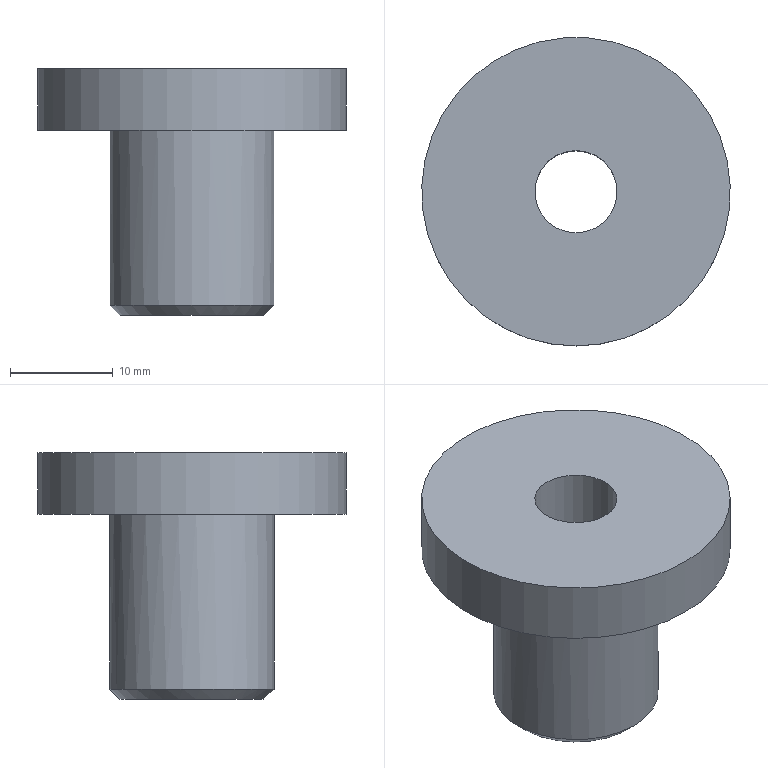Component | NX | MOLD_BASE_ASSY | 1 solid | 7 faces | box 30 x 30 x 24 mm | volume 6630 mm3 | cylinder 3 | plane 3 | cone 1 | commonest cylinder face diameters 16 x1 8 x1 30 x1
STEP:
#1=CARTESIAN_POINT('',(0.,0.,0.));
#2=DIRECTION('',(0.,0.,1.));
#3=DIRECTION('',(1.,0.,0.));
#4=AXIS2_PLACEMENT_3D('',#1,#2,#3);
#5=CARTESIAN_POINT('',(-35.,8.,-7.));
#6=VERTEX_POINT('',#5);
#7=CARTESIAN_POINT('',(-35.,-8.,-7.));
#8=VERTEX_POINT('',#7);
#9=CARTESIAN_POINT('',(-35.,0.,-7.));
#10=DIRECTION('',(0.,0.,1.));
#11=DIRECTION('',(0.,1.,0.));
#12=AXIS2_PLACEMENT_3D('',#9,#10,#11);
#13=CIRCLE('',#12,8.);
#14=CARTESIAN_POINT('',(-35.,0.,-8.));
#15=DIRECTION('',(0.,0.,1.));
#16=DIRECTION('',(0.,-1.,0.));
#17=AXIS2_PLACEMENT_3D('',#14,#15,#16);
#18=CYLINDRICAL_SURFACE('',#17,8.);
#19=CARTESIAN_POINT('',(3.142,1.));
#20=DIRECTION('',(1.,0.));
#21=VECTOR('',#20,1.);
#22=LINE('',#19,#21);
#23=(GEOMETRIC_REPRESENTATION_CONTEXT(2)PARAMETRIC_REPRESENTATION_CONTEXT()REPRESENTATION_CONTEXT('',''));
#24=DEFINITIONAL_REPRESENTATION('',(#22),#23);
#25=PCURVE('',#18,#24);
#26=CARTESIAN_POINT('',(-35.,0.,-7.));
#27=DIRECTION('',(0.,0.,1.));
#28=DIRECTION('',(0.,-1.,0.));
#29=AXIS2_PLACEMENT_3D('',#26,#27,#28);
#30=CONICAL_SURFACE('',#29,8.,0.7854);
#31=CARTESIAN_POINT('',(3.142,0.));
#32=DIRECTION('',(1.,0.));
#33=VECTOR('',#32,1.);
#34=LINE('',#31,#33);
#35=(GEOMETRIC_REPRESENTATION_CONTEXT(2)PARAMETRIC_REPRESENTATION_CONTEXT()REPRESENTATION_CONTEXT('',''));
#36=DEFINITIONAL_REPRESENTATION('',(#34),#35);
#37=PCURVE('',#30,#36);
#38=SURFACE_CURVE('',#13,(#25,#37),.PCURVE_S1.);
#39=EDGE_CURVE('',#6,#8,#38,.T.);
#40=ORIENTED_EDGE('',*,*,#39,.T.);
#41=CARTESIAN_POINT('',(-35.,-8.,10.));
#42=VERTEX_POINT('',#41);
#43=CARTESIAN_POINT('',(-35.,-8.,-7.));
#44=CARTESIAN_POINT('',(-35.,-8.,10.));
#45=B_SPLINE_CURVE_WITH_KNOTS('',1,(#43,#44),.UNSPECIFIED.,.F.,.F.,(2,2),(1.,18.),.PIECEWISE_BEZIER_KNOTS.);
#46=CARTESIAN_POINT('',(6.283,0.));
#47=DIRECTION('',(0.,1.));
#48=VECTOR('',#47,1.);
#49=LINE('',#46,#48);
#50=(GEOMETRIC_REPRESENTATION_CONTEXT(2)PARAMETRIC_REPRESENTATION_CONTEXT()REPRESENTATION_CONTEXT('',''));
#51=DEFINITIONAL_REPRESENTATION('',(#49),#50);
#52=PCURVE('',#18,#51);
#53=CARTESIAN_POINT('',(0.,0.));
#54=DIRECTION('',(0.,1.));
#55=VECTOR('',#54,1.);
#56=LINE('',#53,#55);
#57=(GEOMETRIC_REPRESENTATION_CONTEXT(2)PARAMETRIC_REPRESENTATION_CONTEXT()REPRESENTATION_CONTEXT('',''));
#58=DEFINITIONAL_REPRESENTATION('',(#56),#57);
#59=PCURVE('',#18,#58);
#60=SEAM_CURVE('',#45,(#52,#59),.PCURVE_S1.);
#61=EDGE_CURVE('',#8,#42,#60,.T.);
#62=ORIENTED_EDGE('',*,*,#61,.T.);
#63=CARTESIAN_POINT('',(-35.,0.,10.));
#64=DIRECTION('',(0.,0.,1.));
#65=DIRECTION('',(0.,-1.,0.));
#66=AXIS2_PLACEMENT_3D('',#63,#64,#65);
#67=CIRCLE('',#66,8.);
#68=CARTESIAN_POINT('',(0.,18.));
#69=DIRECTION('',(1.,0.));
#70=VECTOR('',#69,1.);
#71=LINE('',#68,#70);
#72=(GEOMETRIC_REPRESENTATION_CONTEXT(2)PARAMETRIC_REPRESENTATION_CONTEXT()REPRESENTATION_CONTEXT('',''));
#73=DEFINITIONAL_REPRESENTATION('',(#71),#72);
#74=PCURVE('',#18,#73);
#75=CARTESIAN_POINT('',(-35.,15.,10.));
#76=DIRECTION('',(0.,0.,-1.));
#77=DIRECTION('',(0.,1.,0.));
#78=AXIS2_PLACEMENT_3D('',#75,#76,#77);
#79=PLANE('',#78);
#80=CARTESIAN_POINT('',(-23.,0.));
#81=CARTESIAN_POINT('',(-23.,13.856));
#82=CARTESIAN_POINT('',(-11.,6.928));
#83=CARTESIAN_POINT('',(1.,0.));
#84=CARTESIAN_POINT('',(-11.,-6.928));
#85=CARTESIAN_POINT('',(-23.,-13.856));
#86=CARTESIAN_POINT('',(-23.,0.));
#87=(BOUNDED_CURVE()B_SPLINE_CURVE(2,(#80,#81,#82,#83,#84,#85,#86),.UNSPECIFIED.,.T.,.F.)B_SPLINE_CURVE_WITH_KNOTS((1,2,2,2,2,1),(-2.094,0.,2.094,4.189,6.283,8.378),.UNSPECIFIED.)CURVE()GEOMETRIC_REPRESENTATION_ITEM()RATIONAL_B_SPLINE_CURVE((1.,0.5,1.,0.5,1.,0.5,1.))REPRESENTATION_ITEM(''));
#88=(GEOMETRIC_REPRESENTATION_CONTEXT(2)PARAMETRIC_REPRESENTATION_CONTEXT()REPRESENTATION_CONTEXT('',''));
#89=DEFINITIONAL_REPRESENTATION('',(#87),#88);
#90=PCURVE('',#79,#89);
#91=SURFACE_CURVE('',#67,(#74,#90),.PCURVE_S1.);
#92=EDGE_CURVE('',#42,#42,#91,.T.);
#93=ORIENTED_EDGE('',*,*,#92,.F.);
#94=ORIENTED_EDGE('',*,*,#61,.F.);
#95=CARTESIAN_POINT('',(-35.,0.,-7.));
#96=DIRECTION('',(0.,0.,1.));
#97=DIRECTION('',(0.,1.,0.));
#98=AXIS2_PLACEMENT_3D('',#95,#96,#97);
#99=CIRCLE('',#98,8.);
#100=CARTESIAN_POINT('',(-3.142,1.));
#101=DIRECTION('',(1.,0.));
#102=VECTOR('',#101,1.);
#103=LINE('',#100,#102);
#104=(GEOMETRIC_REPRESENTATION_CONTEXT(2)PARAMETRIC_REPRESENTATION_CONTEXT()REPRESENTATION_CONTEXT('',''));
#105=DEFINITIONAL_REPRESENTATION('',(#103),#104);
#106=PCURVE('',#18,#105);
#107=CARTESIAN_POINT('',(3.142,0.));
#108=DIRECTION('',(1.,0.));
#109=VECTOR('',#108,1.);
#110=LINE('',#107,#109);
#111=(GEOMETRIC_REPRESENTATION_CONTEXT(2)PARAMETRIC_REPRESENTATION_CONTEXT()REPRESENTATION_CONTEXT('',''));
#112=DEFINITIONAL_REPRESENTATION('',(#110),#111);
#113=PCURVE('',#30,#112);
#114=SURFACE_CURVE('',#99,(#106,#113),.PCURVE_S1.);
#115=EDGE_CURVE('',#8,#6,#114,.T.);
#116=ORIENTED_EDGE('',*,*,#115,.T.);
#117=EDGE_LOOP('',(#40,#62,#93,#94,#116));
#118=FACE_BOUND('',#117,.T.);
#119=ADVANCED_FACE('',(#118),#18,.T.);
#120=CARTESIAN_POINT('',(-35.,7.,-8.));
#121=VERTEX_POINT('',#120);
#122=CARTESIAN_POINT('',(-35.,0.,-8.));
#123=DIRECTION('',(0.,0.,-1.));
#124=DIRECTION('',(0.,1.,0.));
#125=AXIS2_PLACEMENT_3D('',#122,#123,#124);
#126=CIRCLE('',#125,7.);
#127=CARTESIAN_POINT('',(-35.,8.,-8.));
#128=DIRECTION('',(0.,0.,-1.));
#129=DIRECTION('',(0.,1.,0.));
#130=AXIS2_PLACEMENT_3D('',#127,#128,#129);
#131=PLANE('',#130);
#132=CARTESIAN_POINT('',(-8.,0.));
#133=DIRECTION('',(1.,0.));
#134=AXIS2_PLACEMENT_2D('',#132,#133);
#135=CIRCLE('',#134,7.);
#136=(GEOMETRIC_REPRESENTATION_CONTEXT(2)PARAMETRIC_REPRESENTATION_CONTEXT()REPRESENTATION_CONTEXT('',''));
#137=DEFINITIONAL_REPRESENTATION('',(#135),#136);
#138=PCURVE('',#131,#137);
#139=CARTESIAN_POINT('',(9.425,-1.));
#140=DIRECTION('',(-1.,0.));
#141=VECTOR('',#140,1.);
#142=LINE('',#139,#141);
#143=(GEOMETRIC_REPRESENTATION_CONTEXT(2)PARAMETRIC_REPRESENTATION_CONTEXT()REPRESENTATION_CONTEXT('',''));
#144=DEFINITIONAL_REPRESENTATION('',(#142),#143);
#145=PCURVE('',#30,#144);
#146=SURFACE_CURVE('',#126,(#138,#145),.PCURVE_S1.);
#147=EDGE_CURVE('',#121,#121,#146,.T.);
#148=ORIENTED_EDGE('',*,*,#147,.T.);
#149=EDGE_LOOP('',(#148));
#150=FACE_BOUND('',#149,.T.);
#151=CARTESIAN_POINT('',(-35.,-4.,-8.));
#152=VERTEX_POINT('',#151);
#153=CARTESIAN_POINT('',(-35.,0.,-8.));
#154=DIRECTION('',(0.,0.,1.));
#155=DIRECTION('',(0.,-1.,0.));
#156=AXIS2_PLACEMENT_3D('',#153,#154,#155);
#157=CIRCLE('',#156,4.);
#158=CARTESIAN_POINT('',(-12.,0.));
#159=CARTESIAN_POINT('',(-12.,6.928));
#160=CARTESIAN_POINT('',(-6.,3.464));
#161=CARTESIAN_POINT('',(0.,0.));
#162=CARTESIAN_POINT('',(-6.,-3.464));
#163=CARTESIAN_POINT('',(-12.,-6.928));
#164=CARTESIAN_POINT('',(-12.,0.));
#165=(BOUNDED_CURVE()B_SPLINE_CURVE(2,(#158,#159,#160,#161,#162,#163,#164),.UNSPECIFIED.,.T.,.F.)B_SPLINE_CURVE_WITH_KNOTS((1,2,2,2,2,1),(-2.094,0.,2.094,4.189,6.283,8.378),.UNSPECIFIED.)CURVE()GEOMETRIC_REPRESENTATION_ITEM()RATIONAL_B_SPLINE_CURVE((1.,0.5,1.,0.5,1.,0.5,1.))REPRESENTATION_ITEM(''));
#166=(GEOMETRIC_REPRESENTATION_CONTEXT(2)PARAMETRIC_REPRESENTATION_CONTEXT()REPRESENTATION_CONTEXT('',''));
#167=DEFINITIONAL_REPRESENTATION('',(#165),#166);
#168=PCURVE('',#131,#167);
#169=CARTESIAN_POINT('',(-35.,0.,-8.));
#170=DIRECTION('',(0.,0.,1.));
#171=DIRECTION('',(0.,-1.,0.));
#172=AXIS2_PLACEMENT_3D('',#169,#170,#171);
#173=CYLINDRICAL_SURFACE('',#172,4.);
#174=CARTESIAN_POINT('',(0.,0.));
#175=DIRECTION('',(1.,0.));
#176=VECTOR('',#175,1.);
#177=LINE('',#174,#176);
#178=(GEOMETRIC_REPRESENTATION_CONTEXT(2)PARAMETRIC_REPRESENTATION_CONTEXT()REPRESENTATION_CONTEXT('',''));
#179=DEFINITIONAL_REPRESENTATION('',(#177),#178);
#180=PCURVE('',#173,#179);
#181=SURFACE_CURVE('',#157,(#168,#180),.PCURVE_S1.);
#182=EDGE_CURVE('',#152,#152,#181,.T.);
#183=ORIENTED_EDGE('',*,*,#182,.T.);
#184=EDGE_LOOP('',(#183));
#185=FACE_BOUND('',#184,.T.);
#186=ADVANCED_FACE('',(#150,#185),#131,.T.);
#187=CARTESIAN_POINT('',(-35.,-4.,16.));
#188=VERTEX_POINT('',#187);
#189=CARTESIAN_POINT('',(-35.,0.,16.));
#190=DIRECTION('',(0.,0.,1.));
#191=DIRECTION('',(0.,-1.,0.));
#192=AXIS2_PLACEMENT_3D('',#189,#190,#191);
#193=CIRCLE('',#192,4.);
#194=CARTESIAN_POINT('',(0.,24.));
#195=DIRECTION('',(1.,0.));
#196=VECTOR('',#195,1.);
#197=LINE('',#194,#196);
#198=(GEOMETRIC_REPRESENTATION_CONTEXT(2)PARAMETRIC_REPRESENTATION_CONTEXT()REPRESENTATION_CONTEXT('',''));
#199=DEFINITIONAL_REPRESENTATION('',(#197),#198);
#200=PCURVE('',#173,#199);
#201=CARTESIAN_POINT('',(-35.,4.,16.));
#202=DIRECTION('',(0.,0.,1.));
#203=DIRECTION('',(0.,-1.,0.));
#204=AXIS2_PLACEMENT_3D('',#201,#202,#203);
#205=PLANE('',#204);
#206=CARTESIAN_POINT('',(4.,0.));
#207=DIRECTION('',(1.,0.));
#208=AXIS2_PLACEMENT_2D('',#206,#207);
#209=CIRCLE('',#208,4.);
#210=(GEOMETRIC_REPRESENTATION_CONTEXT(2)PARAMETRIC_REPRESENTATION_CONTEXT()REPRESENTATION_CONTEXT('',''));
#211=DEFINITIONAL_REPRESENTATION('',(#209),#210);
#212=PCURVE('',#205,#211);
#213=SURFACE_CURVE('',#193,(#200,#212),.PCURVE_S1.);
#214=EDGE_CURVE('',#188,#188,#213,.T.);
#215=ORIENTED_EDGE('',*,*,#214,.F.);
#216=CARTESIAN_POINT('',(-35.,-4.,-8.));
#217=CARTESIAN_POINT('',(-35.,-4.,16.));
#218=B_SPLINE_CURVE_WITH_KNOTS('',1,(#216,#217),.UNSPECIFIED.,.F.,.F.,(2,2),(0.,24.),.PIECEWISE_BEZIER_KNOTS.);
#219=CARTESIAN_POINT('',(0.,0.));
#220=DIRECTION('',(0.,1.));
#221=VECTOR('',#220,1.);
#222=LINE('',#219,#221);
#223=(GEOMETRIC_REPRESENTATION_CONTEXT(2)PARAMETRIC_REPRESENTATION_CONTEXT()REPRESENTATION_CONTEXT('',''));
#224=DEFINITIONAL_REPRESENTATION('',(#222),#223);
#225=PCURVE('',#173,#224);
#226=CARTESIAN_POINT('',(6.283,0.));
#227=DIRECTION('',(0.,1.));
#228=VECTOR('',#227,1.);
#229=LINE('',#226,#228);
#230=(GEOMETRIC_REPRESENTATION_CONTEXT(2)PARAMETRIC_REPRESENTATION_CONTEXT()REPRESENTATION_CONTEXT('',''));
#231=DEFINITIONAL_REPRESENTATION('',(#229),#230);
#232=PCURVE('',#173,#231);
#233=SEAM_CURVE('',#218,(#225,#232),.PCURVE_S1.);
#234=EDGE_CURVE('',#152,#188,#233,.T.);
#235=ORIENTED_EDGE('',*,*,#234,.F.);
#236=ORIENTED_EDGE('',*,*,#182,.T.);
#237=ORIENTED_EDGE('',*,*,#234,.T.);
#238=EDGE_LOOP('',(#215,#235,#236,#237));
#239=FACE_BOUND('',#238,.F.);
#240=ADVANCED_FACE('',(#239),#173,.F.);
#241=CARTESIAN_POINT('',(-35.,-15.,16.));
#242=VERTEX_POINT('',#241);
#243=CARTESIAN_POINT('',(-35.,0.,16.));
#244=DIRECTION('',(0.,0.,1.));
#245=DIRECTION('',(0.,-1.,0.));
#246=AXIS2_PLACEMENT_3D('',#243,#244,#245);
#247=CIRCLE('',#246,15.);
#248=CARTESIAN_POINT('',(4.,0.));
#249=DIRECTION('',(1.,0.));
#250=AXIS2_PLACEMENT_2D('',#248,#249);
#251=CIRCLE('',#250,15.);
#252=(GEOMETRIC_REPRESENTATION_CONTEXT(2)PARAMETRIC_REPRESENTATION_CONTEXT()REPRESENTATION_CONTEXT('',''));
#253=DEFINITIONAL_REPRESENTATION('',(#251),#252);
#254=PCURVE('',#205,#253);
#255=CARTESIAN_POINT('',(-35.,0.,-8.));
#256=DIRECTION('',(0.,0.,1.));
#257=DIRECTION('',(0.,-1.,0.));
#258=AXIS2_PLACEMENT_3D('',#255,#256,#257);
#259=CYLINDRICAL_SURFACE('',#258,15.);
#260=CARTESIAN_POINT('',(0.,24.));
#261=DIRECTION('',(1.,0.));
#262=VECTOR('',#261,1.);
#263=LINE('',#260,#262);
#264=(GEOMETRIC_REPRESENTATION_CONTEXT(2)PARAMETRIC_REPRESENTATION_CONTEXT()REPRESENTATION_CONTEXT('',''));
#265=DEFINITIONAL_REPRESENTATION('',(#263),#264);
#266=PCURVE('',#259,#265);
#267=SURFACE_CURVE('',#247,(#254,#266),.PCURVE_S1.);
#268=EDGE_CURVE('',#242,#242,#267,.T.);
#269=ORIENTED_EDGE('',*,*,#268,.T.);
#270=EDGE_LOOP('',(#269));
#271=FACE_BOUND('',#270,.T.);
#272=ORIENTED_EDGE('',*,*,#214,.F.);
#273=EDGE_LOOP('',(#272));
#274=FACE_BOUND('',#273,.T.);
#275=ADVANCED_FACE('',(#271,#274),#205,.T.);
#276=CARTESIAN_POINT('',(-35.,-15.,10.));
#277=VERTEX_POINT('',#276);
#278=CARTESIAN_POINT('',(-35.,0.,10.));
#279=DIRECTION('',(0.,0.,1.));
#280=DIRECTION('',(0.,-1.,0.));
#281=AXIS2_PLACEMENT_3D('',#278,#279,#280);
#282=CIRCLE('',#281,15.);
#283=CARTESIAN_POINT('',(0.,18.));
#284=DIRECTION('',(1.,0.));
#285=VECTOR('',#284,1.);
#286=LINE('',#283,#285);
#287=(GEOMETRIC_REPRESENTATION_CONTEXT(2)PARAMETRIC_REPRESENTATION_CONTEXT()REPRESENTATION_CONTEXT('',''));
#288=DEFINITIONAL_REPRESENTATION('',(#286),#287);
#289=PCURVE('',#259,#288);
#290=CARTESIAN_POINT('',(-30.,0.));
#291=CARTESIAN_POINT('',(-30.,25.981));
#292=CARTESIAN_POINT('',(-7.5,12.99));
#293=CARTESIAN_POINT('',(15.,0.));
#294=CARTESIAN_POINT('',(-7.5,-12.99));
#295=CARTESIAN_POINT('',(-30.,-25.981));
#296=CARTESIAN_POINT('',(-30.,0.));
#297=(BOUNDED_CURVE()B_SPLINE_CURVE(2,(#290,#291,#292,#293,#294,#295,#296),.UNSPECIFIED.,.T.,.F.)B_SPLINE_CURVE_WITH_KNOTS((1,2,2,2,2,1),(-2.094,0.,2.094,4.189,6.283,8.378),.UNSPECIFIED.)CURVE()GEOMETRIC_REPRESENTATION_ITEM()RATIONAL_B_SPLINE_CURVE((1.,0.5,1.,0.5,1.,0.5,1.))REPRESENTATION_ITEM(''));
#298=(GEOMETRIC_REPRESENTATION_CONTEXT(2)PARAMETRIC_REPRESENTATION_CONTEXT()REPRESENTATION_CONTEXT('',''));
#299=DEFINITIONAL_REPRESENTATION('',(#297),#298);
#300=PCURVE('',#79,#299);
#301=SURFACE_CURVE('',#282,(#289,#300),.PCURVE_S1.);
#302=EDGE_CURVE('',#277,#277,#301,.T.);
#303=ORIENTED_EDGE('',*,*,#302,.T.);
#304=CARTESIAN_POINT('',(-35.,-15.,10.));
#305=CARTESIAN_POINT('',(-35.,-15.,16.));
#306=B_SPLINE_CURVE_WITH_KNOTS('',1,(#304,#305),.UNSPECIFIED.,.F.,.F.,(2,2),(18.,24.),.PIECEWISE_BEZIER_KNOTS.);
#307=CARTESIAN_POINT('',(6.283,0.));
#308=DIRECTION('',(0.,1.));
#309=VECTOR('',#308,1.);
#310=LINE('',#307,#309);
#311=(GEOMETRIC_REPRESENTATION_CONTEXT(2)PARAMETRIC_REPRESENTATION_CONTEXT()REPRESENTATION_CONTEXT('',''));
#312=DEFINITIONAL_REPRESENTATION('',(#310),#311);
#313=PCURVE('',#259,#312);
#314=CARTESIAN_POINT('',(0.,0.));
#315=DIRECTION('',(0.,1.));
#316=VECTOR('',#315,1.);
#317=LINE('',#314,#316);
#318=(GEOMETRIC_REPRESENTATION_CONTEXT(2)PARAMETRIC_REPRESENTATION_CONTEXT()REPRESENTATION_CONTEXT('',''));
#319=DEFINITIONAL_REPRESENTATION('',(#317),#318);
#320=PCURVE('',#259,#319);
#321=SEAM_CURVE('',#306,(#313,#320),.PCURVE_S1.);
#322=EDGE_CURVE('',#277,#242,#321,.T.);
#323=ORIENTED_EDGE('',*,*,#322,.T.);
#324=ORIENTED_EDGE('',*,*,#268,.F.);
#325=ORIENTED_EDGE('',*,*,#322,.F.);
#326=EDGE_LOOP('',(#303,#323,#324,#325));
#327=FACE_BOUND('',#326,.T.);
#328=ADVANCED_FACE('',(#327),#259,.T.);
#329=ORIENTED_EDGE('',*,*,#92,.T.);
#330=EDGE_LOOP('',(#329));
#331=FACE_BOUND('',#330,.T.);
#332=ORIENTED_EDGE('',*,*,#302,.F.);
#333=EDGE_LOOP('',(#332));
#334=FACE_BOUND('',#333,.T.);
#335=ADVANCED_FACE('',(#331,#334),#79,.T.);
#336=ORIENTED_EDGE('',*,*,#147,.F.);
#337=CARTESIAN_POINT('',(-35.,7.,-8.));
#338=CARTESIAN_POINT('',(-35.,8.,-7.));
#339=B_SPLINE_CURVE_WITH_KNOTS('',1,(#337,#338),.UNSPECIFIED.,.F.,.F.,(2,2),(-1.414,0.),.PIECEWISE_BEZIER_KNOTS.);
#340=CARTESIAN_POINT('',(9.425,0.));
#341=DIRECTION('',(0.,1.));
#342=VECTOR('',#341,1.);
#343=LINE('',#340,#342);
#344=(GEOMETRIC_REPRESENTATION_CONTEXT(2)PARAMETRIC_REPRESENTATION_CONTEXT()REPRESENTATION_CONTEXT('',''));
#345=DEFINITIONAL_REPRESENTATION('',(#343),#344);
#346=PCURVE('',#30,#345);
#347=CARTESIAN_POINT('',(3.142,0.));
#348=DIRECTION('',(0.,1.));
#349=VECTOR('',#348,1.);
#350=LINE('',#347,#349);
#351=(GEOMETRIC_REPRESENTATION_CONTEXT(2)PARAMETRIC_REPRESENTATION_CONTEXT()REPRESENTATION_CONTEXT('',''));
#352=DEFINITIONAL_REPRESENTATION('',(#350),#351);
#353=PCURVE('',#30,#352);
#354=SEAM_CURVE('',#339,(#346,#353),.PCURVE_S1.);
#355=EDGE_CURVE('',#121,#6,#354,.T.);
#356=ORIENTED_EDGE('',*,*,#355,.T.);
#357=ORIENTED_EDGE('',*,*,#115,.F.);
#358=ORIENTED_EDGE('',*,*,#39,.F.);
#359=ORIENTED_EDGE('',*,*,#355,.F.);
#360=EDGE_LOOP('',(#336,#356,#357,#358,#359));
#361=FACE_BOUND('',#360,.T.);
#362=ADVANCED_FACE('',(#361),#30,.T.);
#363=CLOSED_SHELL('',(#119,#186,#240,#275,#328,#335,#362));
#364=MANIFOLD_SOLID_BREP('',#363);
#365=(LENGTH_UNIT()NAMED_UNIT(*)SI_UNIT(.MILLI.,.METRE.));
#366=UNCERTAINTY_MEASURE_WITH_UNIT(LENGTH_MEASURE(0.00001),#365,'','');
#367=(NAMED_UNIT(*)PLANE_ANGLE_UNIT()SI_UNIT($,.RADIAN.));
#368=(NAMED_UNIT(*)SI_UNIT($,.STERADIAN.)SOLID_ANGLE_UNIT());
#369=(GEOMETRIC_REPRESENTATION_CONTEXT(3)GLOBAL_UNCERTAINTY_ASSIGNED_CONTEXT((#366))GLOBAL_UNIT_ASSIGNED_CONTEXT((#365,#367,#368))REPRESENTATION_CONTEXT('',''));
#370=ADVANCED_BREP_SHAPE_REPRESENTATION('',(#4,#364),#369);